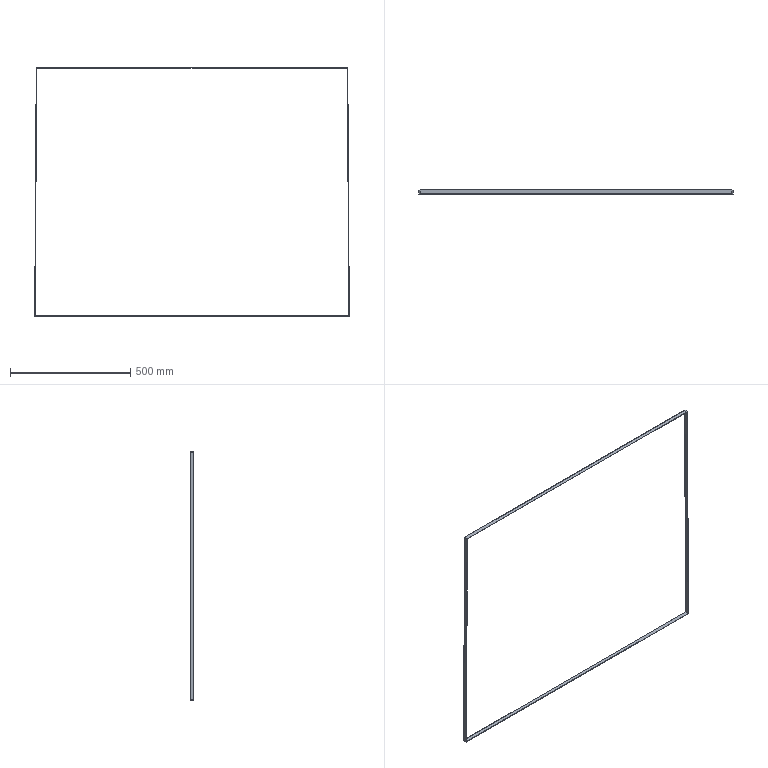Component | NX | LONG_PACKAGING_STRAP | 1 solid | 10 faces | box 1307.7 x 15 x 1031.9 mm | volume 139754 mm3 | plane 10
STEP:
#1=CARTESIAN_POINT('',(0.,0.,0.));
#2=DIRECTION('',(0.,0.,1.));
#3=DIRECTION('',(1.,0.,0.));
#4=AXIS2_PLACEMENT_3D('',#1,#2,#3);
#5=CARTESIAN_POINT('',(-647.456,220.,995.916));
#6=VERTEX_POINT('',#5);
#7=CARTESIAN_POINT('',(647.456,220.,995.916));
#8=VERTEX_POINT('',#7);
#9=CARTESIAN_POINT('',(-645.468,220.,995.916));
#10=DIRECTION('',(1.,0.,0.));
#11=VECTOR('',#10,1.);
#12=LINE('',#9,#11);
#13=CARTESIAN_POINT('',(-645.468,220.,993.916));
#14=DIRECTION('',(0.,1.,0.));
#15=DIRECTION('',(1.,0.,0.));
#16=AXIS2_PLACEMENT_3D('',#13,#14,#15);
#17=PLANE('',#16);
#18=CARTESIAN_POINT('',(0.,-2.));
#19=DIRECTION('',(1.,0.));
#20=VECTOR('',#19,1.);
#21=LINE('',#18,#20);
#22=(GEOMETRIC_REPRESENTATION_CONTEXT(2)PARAMETRIC_REPRESENTATION_CONTEXT()REPRESENTATION_CONTEXT('',''));
#23=DEFINITIONAL_REPRESENTATION('',(#21),#22);
#24=PCURVE('',#17,#23);
#25=CARTESIAN_POINT('',(-645.468,235.,995.916));
#26=DIRECTION('',(0.,0.,-1.));
#27=DIRECTION('',(-1.,0.,0.));
#28=AXIS2_PLACEMENT_3D('',#25,#26,#27);
#29=PLANE('',#28);
#30=CARTESIAN_POINT('',(0.,-15.));
#31=DIRECTION('',(-1.,0.));
#32=VECTOR('',#31,1.);
#33=LINE('',#30,#32);
#34=(GEOMETRIC_REPRESENTATION_CONTEXT(2)PARAMETRIC_REPRESENTATION_CONTEXT()REPRESENTATION_CONTEXT('',''));
#35=DEFINITIONAL_REPRESENTATION('',(#33),#34);
#36=PCURVE('',#29,#35);
#37=SURFACE_CURVE('',#12,(#24,#36),.PCURVE_S1.);
#38=EDGE_CURVE('',#6,#8,#37,.T.);
#39=ORIENTED_EDGE('',*,*,#38,.F.);
#40=CARTESIAN_POINT('',(-653.85,220.,-35.987));
#41=VERTEX_POINT('',#40);
#42=CARTESIAN_POINT('',(-653.838,220.,-33.975));
#43=DIRECTION('',(0.006197,0.,1.));
#44=VECTOR('',#43,1.);
#45=LINE('',#42,#44);
#46=CARTESIAN_POINT('',(-8.37,1027.891));
#47=DIRECTION('',(0.006197,-1.));
#48=VECTOR('',#47,1.);
#49=LINE('',#46,#48);
#50=(GEOMETRIC_REPRESENTATION_CONTEXT(2)PARAMETRIC_REPRESENTATION_CONTEXT()REPRESENTATION_CONTEXT('',''));
#51=DEFINITIONAL_REPRESENTATION('',(#49),#50);
#52=PCURVE('',#17,#51);
#53=CARTESIAN_POINT('',(-653.838,235.,-33.975));
#54=DIRECTION('',(1.,0.,-0.006197));
#55=DIRECTION('',(-0.006197,0.,-1.));
#56=AXIS2_PLACEMENT_3D('',#53,#54,#55);
#57=PLANE('',#56);
#58=CARTESIAN_POINT('',(0.,-15.));
#59=DIRECTION('',(-1.,0.));
#60=VECTOR('',#59,1.);
#61=LINE('',#58,#60);
#62=(GEOMETRIC_REPRESENTATION_CONTEXT(2)PARAMETRIC_REPRESENTATION_CONTEXT()REPRESENTATION_CONTEXT('',''));
#63=DEFINITIONAL_REPRESENTATION('',(#61),#62);
#64=PCURVE('',#57,#63);
#65=SURFACE_CURVE('',#45,(#52,#64),.PCURVE_S1.);
#66=EDGE_CURVE('',#41,#6,#65,.T.);
#67=ORIENTED_EDGE('',*,*,#66,.F.);
#68=CARTESIAN_POINT('',(653.85,220.,-35.987));
#69=VERTEX_POINT('',#68);
#70=CARTESIAN_POINT('',(651.838,220.,-35.987));
#71=DIRECTION('',(-1.,0.,-0.));
#72=VECTOR('',#71,1.);
#73=LINE('',#70,#72);
#74=CARTESIAN_POINT('',(1297.306,1029.903));
#75=DIRECTION('',(-1.,0.));
#76=VECTOR('',#75,1.);
#77=LINE('',#74,#76);
#78=(GEOMETRIC_REPRESENTATION_CONTEXT(2)PARAMETRIC_REPRESENTATION_CONTEXT()REPRESENTATION_CONTEXT('',''));
#79=DEFINITIONAL_REPRESENTATION('',(#77),#78);
#80=PCURVE('',#17,#79);
#81=CARTESIAN_POINT('',(651.838,235.,-35.987));
#82=DIRECTION('',(-0.,0.,1.));
#83=DIRECTION('',(1.,0.,0.));
#84=AXIS2_PLACEMENT_3D('',#81,#82,#83);
#85=PLANE('',#84);
#86=CARTESIAN_POINT('',(0.,-15.));
#87=DIRECTION('',(-1.,0.));
#88=VECTOR('',#87,1.);
#89=LINE('',#86,#88);
#90=(GEOMETRIC_REPRESENTATION_CONTEXT(2)PARAMETRIC_REPRESENTATION_CONTEXT()REPRESENTATION_CONTEXT('',''));
#91=DEFINITIONAL_REPRESENTATION('',(#89),#90);
#92=PCURVE('',#85,#91);
#93=SURFACE_CURVE('',#73,(#80,#92),.PCURVE_S1.);
#94=EDGE_CURVE('',#69,#41,#93,.T.);
#95=ORIENTED_EDGE('',*,*,#94,.F.);
#96=CARTESIAN_POINT('',(647.468,220.,993.928));
#97=DIRECTION('',(0.006197,0.,-1.));
#98=VECTOR('',#97,1.);
#99=LINE('',#96,#98);
#100=CARTESIAN_POINT('',(1292.936,-0.01239));
#101=DIRECTION('',(0.006197,1.));
#102=VECTOR('',#101,1.);
#103=LINE('',#100,#102);
#104=(GEOMETRIC_REPRESENTATION_CONTEXT(2)PARAMETRIC_REPRESENTATION_CONTEXT()REPRESENTATION_CONTEXT('',''));
#105=DEFINITIONAL_REPRESENTATION('',(#103),#104);
#106=PCURVE('',#17,#105);
#107=CARTESIAN_POINT('',(647.468,235.,993.928));
#108=DIRECTION('',(-1.,0.,-0.006197));
#109=DIRECTION('',(-0.006197,0.,1.));
#110=AXIS2_PLACEMENT_3D('',#107,#108,#109);
#111=PLANE('',#110);
#112=CARTESIAN_POINT('',(0.,-15.));
#113=DIRECTION('',(-1.,0.));
#114=VECTOR('',#113,1.);
#115=LINE('',#112,#114);
#116=(GEOMETRIC_REPRESENTATION_CONTEXT(2)PARAMETRIC_REPRESENTATION_CONTEXT()REPRESENTATION_CONTEXT('',''));
#117=DEFINITIONAL_REPRESENTATION('',(#115),#116);
#118=PCURVE('',#111,#117);
#119=SURFACE_CURVE('',#99,(#106,#118),.PCURVE_S1.);
#120=EDGE_CURVE('',#8,#69,#119,.T.);
#121=ORIENTED_EDGE('',*,*,#120,.F.);
#122=EDGE_LOOP('',(#39,#67,#95,#121));
#123=FACE_BOUND('',#122,.T.);
#124=CARTESIAN_POINT('',(-645.468,220.,993.916));
#125=VERTEX_POINT('',#124);
#126=CARTESIAN_POINT('',(645.468,220.,993.916));
#127=VERTEX_POINT('',#126);
#128=CARTESIAN_POINT('',(-645.468,220.,993.916));
#129=DIRECTION('',(1.,0.,0.));
#130=VECTOR('',#129,1.);
#131=LINE('',#128,#130);
#132=CARTESIAN_POINT('',(0.,0.));
#133=DIRECTION('',(1.,0.));
#134=VECTOR('',#133,1.);
#135=LINE('',#132,#134);
#136=(GEOMETRIC_REPRESENTATION_CONTEXT(2)PARAMETRIC_REPRESENTATION_CONTEXT()REPRESENTATION_CONTEXT('',''));
#137=DEFINITIONAL_REPRESENTATION('',(#135),#136);
#138=PCURVE('',#17,#137);
#139=CARTESIAN_POINT('',(-645.468,235.,993.916));
#140=DIRECTION('',(0.,0.,-1.));
#141=DIRECTION('',(-1.,0.,0.));
#142=AXIS2_PLACEMENT_3D('',#139,#140,#141);
#143=PLANE('',#142);
#144=CARTESIAN_POINT('',(0.,-15.));
#145=DIRECTION('',(-1.,0.));
#146=VECTOR('',#145,1.);
#147=LINE('',#144,#146);
#148=(GEOMETRIC_REPRESENTATION_CONTEXT(2)PARAMETRIC_REPRESENTATION_CONTEXT()REPRESENTATION_CONTEXT('',''));
#149=DEFINITIONAL_REPRESENTATION('',(#147),#148);
#150=PCURVE('',#143,#149);
#151=SURFACE_CURVE('',#131,(#138,#150),.PCURVE_S1.);
#152=EDGE_CURVE('',#125,#127,#151,.T.);
#153=ORIENTED_EDGE('',*,*,#152,.T.);
#154=CARTESIAN_POINT('',(651.838,220.,-33.987));
#155=VERTEX_POINT('',#154);
#156=CARTESIAN_POINT('',(645.468,220.,993.916));
#157=DIRECTION('',(0.006197,0.,-1.));
#158=VECTOR('',#157,1.);
#159=LINE('',#156,#158);
#160=CARTESIAN_POINT('',(1290.936,0.));
#161=DIRECTION('',(0.006197,1.));
#162=VECTOR('',#161,1.);
#163=LINE('',#160,#162);
#164=(GEOMETRIC_REPRESENTATION_CONTEXT(2)PARAMETRIC_REPRESENTATION_CONTEXT()REPRESENTATION_CONTEXT('',''));
#165=DEFINITIONAL_REPRESENTATION('',(#163),#164);
#166=PCURVE('',#17,#165);
#167=CARTESIAN_POINT('',(645.468,235.,993.916));
#168=DIRECTION('',(-1.,0.,-0.006197));
#169=DIRECTION('',(-0.006197,0.,1.));
#170=AXIS2_PLACEMENT_3D('',#167,#168,#169);
#171=PLANE('',#170);
#172=CARTESIAN_POINT('',(0.,-15.));
#173=DIRECTION('',(-1.,0.));
#174=VECTOR('',#173,1.);
#175=LINE('',#172,#174);
#176=(GEOMETRIC_REPRESENTATION_CONTEXT(2)PARAMETRIC_REPRESENTATION_CONTEXT()REPRESENTATION_CONTEXT('',''));
#177=DEFINITIONAL_REPRESENTATION('',(#175),#176);
#178=PCURVE('',#171,#177);
#179=SURFACE_CURVE('',#159,(#166,#178),.PCURVE_S1.);
#180=EDGE_CURVE('',#127,#155,#179,.T.);
#181=ORIENTED_EDGE('',*,*,#180,.T.);
#182=CARTESIAN_POINT('',(-651.838,220.,-33.987));
#183=VERTEX_POINT('',#182);
#184=CARTESIAN_POINT('',(651.838,220.,-33.987));
#185=DIRECTION('',(-1.,0.,-0.));
#186=VECTOR('',#185,1.);
#187=LINE('',#184,#186);
#188=CARTESIAN_POINT('',(1297.306,1027.903));
#189=DIRECTION('',(-1.,0.));
#190=VECTOR('',#189,1.);
#191=LINE('',#188,#190);
#192=(GEOMETRIC_REPRESENTATION_CONTEXT(2)PARAMETRIC_REPRESENTATION_CONTEXT()REPRESENTATION_CONTEXT('',''));
#193=DEFINITIONAL_REPRESENTATION('',(#191),#192);
#194=PCURVE('',#17,#193);
#195=CARTESIAN_POINT('',(651.838,235.,-33.987));
#196=DIRECTION('',(-0.,0.,1.));
#197=DIRECTION('',(1.,0.,0.));
#198=AXIS2_PLACEMENT_3D('',#195,#196,#197);
#199=PLANE('',#198);
#200=CARTESIAN_POINT('',(0.,-15.));
#201=DIRECTION('',(-1.,0.));
#202=VECTOR('',#201,1.);
#203=LINE('',#200,#202);
#204=(GEOMETRIC_REPRESENTATION_CONTEXT(2)PARAMETRIC_REPRESENTATION_CONTEXT()REPRESENTATION_CONTEXT('',''));
#205=DEFINITIONAL_REPRESENTATION('',(#203),#204);
#206=PCURVE('',#199,#205);
#207=SURFACE_CURVE('',#187,(#194,#206),.PCURVE_S1.);
#208=EDGE_CURVE('',#155,#183,#207,.T.);
#209=ORIENTED_EDGE('',*,*,#208,.T.);
#210=CARTESIAN_POINT('',(-651.838,220.,-33.987));
#211=DIRECTION('',(0.006197,0.,1.));
#212=VECTOR('',#211,1.);
#213=LINE('',#210,#212);
#214=CARTESIAN_POINT('',(-6.37,1027.903));
#215=DIRECTION('',(0.006197,-1.));
#216=VECTOR('',#215,1.);
#217=LINE('',#214,#216);
#218=(GEOMETRIC_REPRESENTATION_CONTEXT(2)PARAMETRIC_REPRESENTATION_CONTEXT()REPRESENTATION_CONTEXT('',''));
#219=DEFINITIONAL_REPRESENTATION('',(#217),#218);
#220=PCURVE('',#17,#219);
#221=CARTESIAN_POINT('',(-651.838,235.,-33.987));
#222=DIRECTION('',(1.,0.,-0.006197));
#223=DIRECTION('',(-0.006197,0.,-1.));
#224=AXIS2_PLACEMENT_3D('',#221,#222,#223);
#225=PLANE('',#224);
#226=CARTESIAN_POINT('',(0.,-15.));
#227=DIRECTION('',(-1.,0.));
#228=VECTOR('',#227,1.);
#229=LINE('',#226,#228);
#230=(GEOMETRIC_REPRESENTATION_CONTEXT(2)PARAMETRIC_REPRESENTATION_CONTEXT()REPRESENTATION_CONTEXT('',''));
#231=DEFINITIONAL_REPRESENTATION('',(#229),#230);
#232=PCURVE('',#225,#231);
#233=SURFACE_CURVE('',#213,(#220,#232),.PCURVE_S1.);
#234=EDGE_CURVE('',#183,#125,#233,.T.);
#235=ORIENTED_EDGE('',*,*,#234,.T.);
#236=EDGE_LOOP('',(#153,#181,#209,#235));
#237=FACE_BOUND('',#236,.T.);
#238=ADVANCED_FACE('',(#123,#237),#17,.F.);
#239=CARTESIAN_POINT('',(653.85,235.,-35.987));
#240=VERTEX_POINT('',#239);
#241=CARTESIAN_POINT('',(-653.85,235.,-35.987));
#242=VERTEX_POINT('',#241);
#243=CARTESIAN_POINT('',(651.838,235.,-35.987));
#244=DIRECTION('',(-1.,0.,-0.));
#245=VECTOR('',#244,1.);
#246=LINE('',#243,#245);
#247=CARTESIAN_POINT('',(651.838,235.,-33.987));
#248=DIRECTION('',(0.,1.,0.));
#249=DIRECTION('',(-1.,0.,-0.));
#250=AXIS2_PLACEMENT_3D('',#247,#248,#249);
#251=PLANE('',#250);
#252=CARTESIAN_POINT('',(0.,-2.));
#253=DIRECTION('',(1.,-0.));
#254=VECTOR('',#253,1.);
#255=LINE('',#252,#254);
#256=(GEOMETRIC_REPRESENTATION_CONTEXT(2)PARAMETRIC_REPRESENTATION_CONTEXT()REPRESENTATION_CONTEXT('',''));
#257=DEFINITIONAL_REPRESENTATION('',(#255),#256);
#258=PCURVE('',#251,#257);
#259=CARTESIAN_POINT('',(0.,0.));
#260=DIRECTION('',(-1.,0.));
#261=VECTOR('',#260,1.);
#262=LINE('',#259,#261);
#263=(GEOMETRIC_REPRESENTATION_CONTEXT(2)PARAMETRIC_REPRESENTATION_CONTEXT()REPRESENTATION_CONTEXT('',''));
#264=DEFINITIONAL_REPRESENTATION('',(#262),#263);
#265=PCURVE('',#85,#264);
#266=SURFACE_CURVE('',#246,(#258,#265),.PCURVE_S1.);
#267=EDGE_CURVE('',#240,#242,#266,.T.);
#268=ORIENTED_EDGE('',*,*,#267,.T.);
#269=CARTESIAN_POINT('',(-647.456,235.,995.916));
#270=VERTEX_POINT('',#269);
#271=CARTESIAN_POINT('',(-653.838,235.,-33.975));
#272=DIRECTION('',(0.006197,0.,1.));
#273=VECTOR('',#272,1.);
#274=LINE('',#271,#273);
#275=CARTESIAN_POINT('',(1305.676,0.01239));
#276=DIRECTION('',(-0.006197,1.));
#277=VECTOR('',#276,1.);
#278=LINE('',#275,#277);
#279=(GEOMETRIC_REPRESENTATION_CONTEXT(2)PARAMETRIC_REPRESENTATION_CONTEXT()REPRESENTATION_CONTEXT('',''));
#280=DEFINITIONAL_REPRESENTATION('',(#278),#279);
#281=PCURVE('',#251,#280);
#282=CARTESIAN_POINT('',(0.,0.));
#283=DIRECTION('',(-1.,0.));
#284=VECTOR('',#283,1.);
#285=LINE('',#282,#284);
#286=(GEOMETRIC_REPRESENTATION_CONTEXT(2)PARAMETRIC_REPRESENTATION_CONTEXT()REPRESENTATION_CONTEXT('',''));
#287=DEFINITIONAL_REPRESENTATION('',(#285),#286);
#288=PCURVE('',#57,#287);
#289=SURFACE_CURVE('',#274,(#281,#288),.PCURVE_S1.);
#290=EDGE_CURVE('',#242,#270,#289,.T.);
#291=ORIENTED_EDGE('',*,*,#290,.T.);
#292=CARTESIAN_POINT('',(647.456,235.,995.916));
#293=VERTEX_POINT('',#292);
#294=CARTESIAN_POINT('',(-645.468,235.,995.916));
#295=DIRECTION('',(1.,0.,0.));
#296=VECTOR('',#295,1.);
#297=LINE('',#294,#296);
#298=CARTESIAN_POINT('',(1297.306,1029.903));
#299=DIRECTION('',(-1.,-0.));
#300=VECTOR('',#299,1.);
#301=LINE('',#298,#300);
#302=(GEOMETRIC_REPRESENTATION_CONTEXT(2)PARAMETRIC_REPRESENTATION_CONTEXT()REPRESENTATION_CONTEXT('',''));
#303=DEFINITIONAL_REPRESENTATION('',(#301),#302);
#304=PCURVE('',#251,#303);
#305=CARTESIAN_POINT('',(0.,0.));
#306=DIRECTION('',(-1.,0.));
#307=VECTOR('',#306,1.);
#308=LINE('',#305,#307);
#309=(GEOMETRIC_REPRESENTATION_CONTEXT(2)PARAMETRIC_REPRESENTATION_CONTEXT()REPRESENTATION_CONTEXT('',''));
#310=DEFINITIONAL_REPRESENTATION('',(#308),#309);
#311=PCURVE('',#29,#310);
#312=SURFACE_CURVE('',#297,(#304,#311),.PCURVE_S1.);
#313=EDGE_CURVE('',#270,#293,#312,.T.);
#314=ORIENTED_EDGE('',*,*,#313,.T.);
#315=CARTESIAN_POINT('',(647.468,235.,993.928));
#316=DIRECTION('',(0.006197,0.,-1.));
#317=VECTOR('',#316,1.);
#318=LINE('',#315,#317);
#319=CARTESIAN_POINT('',(4.37,1027.915));
#320=DIRECTION('',(-0.006197,-1.));
#321=VECTOR('',#320,1.);
#322=LINE('',#319,#321);
#323=(GEOMETRIC_REPRESENTATION_CONTEXT(2)PARAMETRIC_REPRESENTATION_CONTEXT()REPRESENTATION_CONTEXT('',''));
#324=DEFINITIONAL_REPRESENTATION('',(#322),#323);
#325=PCURVE('',#251,#324);
#326=CARTESIAN_POINT('',(0.,0.));
#327=DIRECTION('',(-1.,0.));
#328=VECTOR('',#327,1.);
#329=LINE('',#326,#328);
#330=(GEOMETRIC_REPRESENTATION_CONTEXT(2)PARAMETRIC_REPRESENTATION_CONTEXT()REPRESENTATION_CONTEXT('',''));
#331=DEFINITIONAL_REPRESENTATION('',(#329),#330);
#332=PCURVE('',#111,#331);
#333=SURFACE_CURVE('',#318,(#325,#332),.PCURVE_S1.);
#334=EDGE_CURVE('',#293,#240,#333,.T.);
#335=ORIENTED_EDGE('',*,*,#334,.T.);
#336=EDGE_LOOP('',(#268,#291,#314,#335));
#337=FACE_BOUND('',#336,.T.);
#338=CARTESIAN_POINT('',(651.838,235.,-33.987));
#339=VERTEX_POINT('',#338);
#340=CARTESIAN_POINT('',(-651.838,235.,-33.987));
#341=VERTEX_POINT('',#340);
#342=CARTESIAN_POINT('',(651.838,235.,-33.987));
#343=DIRECTION('',(-1.,0.,-0.));
#344=VECTOR('',#343,1.);
#345=LINE('',#342,#344);
#346=CARTESIAN_POINT('',(0.,0.));
#347=DIRECTION('',(1.,-0.));
#348=VECTOR('',#347,1.);
#349=LINE('',#346,#348);
#350=(GEOMETRIC_REPRESENTATION_CONTEXT(2)PARAMETRIC_REPRESENTATION_CONTEXT()REPRESENTATION_CONTEXT('',''));
#351=DEFINITIONAL_REPRESENTATION('',(#349),#350);
#352=PCURVE('',#251,#351);
#353=CARTESIAN_POINT('',(0.,0.));
#354=DIRECTION('',(-1.,0.));
#355=VECTOR('',#354,1.);
#356=LINE('',#353,#355);
#357=(GEOMETRIC_REPRESENTATION_CONTEXT(2)PARAMETRIC_REPRESENTATION_CONTEXT()REPRESENTATION_CONTEXT('',''));
#358=DEFINITIONAL_REPRESENTATION('',(#356),#357);
#359=PCURVE('',#199,#358);
#360=SURFACE_CURVE('',#345,(#352,#359),.PCURVE_S1.);
#361=EDGE_CURVE('',#339,#341,#360,.T.);
#362=ORIENTED_EDGE('',*,*,#361,.F.);
#363=CARTESIAN_POINT('',(645.468,235.,993.916));
#364=VERTEX_POINT('',#363);
#365=CARTESIAN_POINT('',(645.468,235.,993.916));
#366=DIRECTION('',(0.006197,0.,-1.));
#367=VECTOR('',#366,1.);
#368=LINE('',#365,#367);
#369=CARTESIAN_POINT('',(6.37,1027.903));
#370=DIRECTION('',(-0.006197,-1.));
#371=VECTOR('',#370,1.);
#372=LINE('',#369,#371);
#373=(GEOMETRIC_REPRESENTATION_CONTEXT(2)PARAMETRIC_REPRESENTATION_CONTEXT()REPRESENTATION_CONTEXT('',''));
#374=DEFINITIONAL_REPRESENTATION('',(#372),#373);
#375=PCURVE('',#251,#374);
#376=CARTESIAN_POINT('',(0.,0.));
#377=DIRECTION('',(-1.,0.));
#378=VECTOR('',#377,1.);
#379=LINE('',#376,#378);
#380=(GEOMETRIC_REPRESENTATION_CONTEXT(2)PARAMETRIC_REPRESENTATION_CONTEXT()REPRESENTATION_CONTEXT('',''));
#381=DEFINITIONAL_REPRESENTATION('',(#379),#380);
#382=PCURVE('',#171,#381);
#383=SURFACE_CURVE('',#368,(#375,#382),.PCURVE_S1.);
#384=EDGE_CURVE('',#364,#339,#383,.T.);
#385=ORIENTED_EDGE('',*,*,#384,.F.);
#386=CARTESIAN_POINT('',(-645.468,235.,993.916));
#387=VERTEX_POINT('',#386);
#388=CARTESIAN_POINT('',(-645.468,235.,993.916));
#389=DIRECTION('',(1.,0.,0.));
#390=VECTOR('',#389,1.);
#391=LINE('',#388,#390);
#392=CARTESIAN_POINT('',(1297.306,1027.903));
#393=DIRECTION('',(-1.,-0.));
#394=VECTOR('',#393,1.);
#395=LINE('',#392,#394);
#396=(GEOMETRIC_REPRESENTATION_CONTEXT(2)PARAMETRIC_REPRESENTATION_CONTEXT()REPRESENTATION_CONTEXT('',''));
#397=DEFINITIONAL_REPRESENTATION('',(#395),#396);
#398=PCURVE('',#251,#397);
#399=CARTESIAN_POINT('',(0.,0.));
#400=DIRECTION('',(-1.,0.));
#401=VECTOR('',#400,1.);
#402=LINE('',#399,#401);
#403=(GEOMETRIC_REPRESENTATION_CONTEXT(2)PARAMETRIC_REPRESENTATION_CONTEXT()REPRESENTATION_CONTEXT('',''));
#404=DEFINITIONAL_REPRESENTATION('',(#402),#403);
#405=PCURVE('',#143,#404);
#406=SURFACE_CURVE('',#391,(#398,#405),.PCURVE_S1.);
#407=EDGE_CURVE('',#387,#364,#406,.T.);
#408=ORIENTED_EDGE('',*,*,#407,.F.);
#409=CARTESIAN_POINT('',(-651.838,235.,-33.987));
#410=DIRECTION('',(0.006197,0.,1.));
#411=VECTOR('',#410,1.);
#412=LINE('',#409,#411);
#413=CARTESIAN_POINT('',(1303.676,-0.));
#414=DIRECTION('',(-0.006197,1.));
#415=VECTOR('',#414,1.);
#416=LINE('',#413,#415);
#417=(GEOMETRIC_REPRESENTATION_CONTEXT(2)PARAMETRIC_REPRESENTATION_CONTEXT()REPRESENTATION_CONTEXT('',''));
#418=DEFINITIONAL_REPRESENTATION('',(#416),#417);
#419=PCURVE('',#251,#418);
#420=CARTESIAN_POINT('',(0.,0.));
#421=DIRECTION('',(-1.,0.));
#422=VECTOR('',#421,1.);
#423=LINE('',#420,#422);
#424=(GEOMETRIC_REPRESENTATION_CONTEXT(2)PARAMETRIC_REPRESENTATION_CONTEXT()REPRESENTATION_CONTEXT('',''));
#425=DEFINITIONAL_REPRESENTATION('',(#423),#424);
#426=PCURVE('',#225,#425);
#427=SURFACE_CURVE('',#412,(#419,#426),.PCURVE_S1.);
#428=EDGE_CURVE('',#341,#387,#427,.T.);
#429=ORIENTED_EDGE('',*,*,#428,.F.);
#430=EDGE_LOOP('',(#362,#385,#408,#429));
#431=FACE_BOUND('',#430,.T.);
#432=ADVANCED_FACE('',(#337,#431),#251,.T.);
#433=ORIENTED_EDGE('',*,*,#66,.T.);
#434=CARTESIAN_POINT('',(-647.456,235.,995.916));
#435=DIRECTION('',(0.,-1.,0.));
#436=VECTOR('',#435,1.);
#437=LINE('',#434,#436);
#438=CARTESIAN_POINT('',(-1029.91,0.));
#439=DIRECTION('',(0.,-1.));
#440=VECTOR('',#439,1.);
#441=LINE('',#438,#440);
#442=(GEOMETRIC_REPRESENTATION_CONTEXT(2)PARAMETRIC_REPRESENTATION_CONTEXT()REPRESENTATION_CONTEXT('',''));
#443=DEFINITIONAL_REPRESENTATION('',(#441),#442);
#444=PCURVE('',#57,#443);
#445=CARTESIAN_POINT('',(1.988,0.));
#446=DIRECTION('',(0.,-1.));
#447=VECTOR('',#446,1.);
#448=LINE('',#445,#447);
#449=(GEOMETRIC_REPRESENTATION_CONTEXT(2)PARAMETRIC_REPRESENTATION_CONTEXT()REPRESENTATION_CONTEXT('',''));
#450=DEFINITIONAL_REPRESENTATION('',(#448),#449);
#451=PCURVE('',#29,#450);
#452=SURFACE_CURVE('',#437,(#444,#451),.PCURVE_S1.);
#453=EDGE_CURVE('',#270,#6,#452,.T.);
#454=ORIENTED_EDGE('',*,*,#453,.F.);
#455=ORIENTED_EDGE('',*,*,#290,.F.);
#456=CARTESIAN_POINT('',(-653.85,235.,-35.987));
#457=DIRECTION('',(0.,-1.,0.));
#458=VECTOR('',#457,1.);
#459=LINE('',#456,#458);
#460=CARTESIAN_POINT('',(2.012,0.));
#461=DIRECTION('',(0.,-1.));
#462=VECTOR('',#461,1.);
#463=LINE('',#460,#462);
#464=(GEOMETRIC_REPRESENTATION_CONTEXT(2)PARAMETRIC_REPRESENTATION_CONTEXT()REPRESENTATION_CONTEXT('',''));
#465=DEFINITIONAL_REPRESENTATION('',(#463),#464);
#466=PCURVE('',#57,#465);
#467=CARTESIAN_POINT('',(-1305.689,0.));
#468=DIRECTION('',(0.,-1.));
#469=VECTOR('',#468,1.);
#470=LINE('',#467,#469);
#471=(GEOMETRIC_REPRESENTATION_CONTEXT(2)PARAMETRIC_REPRESENTATION_CONTEXT()REPRESENTATION_CONTEXT('',''));
#472=DEFINITIONAL_REPRESENTATION('',(#470),#471);
#473=PCURVE('',#85,#472);
#474=SURFACE_CURVE('',#459,(#466,#473),.PCURVE_S1.);
#475=EDGE_CURVE('',#242,#41,#474,.T.);
#476=ORIENTED_EDGE('',*,*,#475,.T.);
#477=EDGE_LOOP('',(#433,#454,#455,#476));
#478=FACE_BOUND('',#477,.T.);
#479=ADVANCED_FACE('',(#478),#57,.F.);
#480=ORIENTED_EDGE('',*,*,#38,.T.);
#481=CARTESIAN_POINT('',(647.456,235.,995.916));
#482=DIRECTION('',(0.,-1.,0.));
#483=VECTOR('',#482,1.);
#484=LINE('',#481,#483);
#485=CARTESIAN_POINT('',(-1292.924,0.));
#486=DIRECTION('',(0.,-1.));
#487=VECTOR('',#486,1.);
#488=LINE('',#485,#487);
#489=(GEOMETRIC_REPRESENTATION_CONTEXT(2)PARAMETRIC_REPRESENTATION_CONTEXT()REPRESENTATION_CONTEXT('',''));
#490=DEFINITIONAL_REPRESENTATION('',(#488),#489);
#491=PCURVE('',#29,#490);
#492=CARTESIAN_POINT('',(1.988,0.));
#493=DIRECTION('',(0.,-1.));
#494=VECTOR('',#493,1.);
#495=LINE('',#492,#494);
#496=(GEOMETRIC_REPRESENTATION_CONTEXT(2)PARAMETRIC_REPRESENTATION_CONTEXT()REPRESENTATION_CONTEXT('',''));
#497=DEFINITIONAL_REPRESENTATION('',(#495),#496);
#498=PCURVE('',#111,#497);
#499=SURFACE_CURVE('',#484,(#491,#498),.PCURVE_S1.);
#500=EDGE_CURVE('',#293,#8,#499,.T.);
#501=ORIENTED_EDGE('',*,*,#500,.F.);
#502=ORIENTED_EDGE('',*,*,#313,.F.);
#503=ORIENTED_EDGE('',*,*,#453,.T.);
#504=EDGE_LOOP('',(#480,#501,#502,#503));
#505=FACE_BOUND('',#504,.T.);
#506=ADVANCED_FACE('',(#505),#29,.F.);
#507=ORIENTED_EDGE('',*,*,#120,.T.);
#508=CARTESIAN_POINT('',(653.85,235.,-35.987));
#509=DIRECTION('',(0.,-1.,0.));
#510=VECTOR('',#509,1.);
#511=LINE('',#508,#510);
#512=CARTESIAN_POINT('',(-1029.935,0.));
#513=DIRECTION('',(0.,-1.));
#514=VECTOR('',#513,1.);
#515=LINE('',#512,#514);
#516=(GEOMETRIC_REPRESENTATION_CONTEXT(2)PARAMETRIC_REPRESENTATION_CONTEXT()REPRESENTATION_CONTEXT('',''));
#517=DEFINITIONAL_REPRESENTATION('',(#515),#516);
#518=PCURVE('',#111,#517);
#519=CARTESIAN_POINT('',(2.012,0.));
#520=DIRECTION('',(0.,-1.));
#521=VECTOR('',#520,1.);
#522=LINE('',#519,#521);
#523=(GEOMETRIC_REPRESENTATION_CONTEXT(2)PARAMETRIC_REPRESENTATION_CONTEXT()REPRESENTATION_CONTEXT('',''));
#524=DEFINITIONAL_REPRESENTATION('',(#522),#523);
#525=PCURVE('',#85,#524);
#526=SURFACE_CURVE('',#511,(#518,#525),.PCURVE_S1.);
#527=EDGE_CURVE('',#240,#69,#526,.T.);
#528=ORIENTED_EDGE('',*,*,#527,.F.);
#529=ORIENTED_EDGE('',*,*,#334,.F.);
#530=ORIENTED_EDGE('',*,*,#500,.T.);
#531=EDGE_LOOP('',(#507,#528,#529,#530));
#532=FACE_BOUND('',#531,.T.);
#533=ADVANCED_FACE('',(#532),#111,.F.);
#534=ORIENTED_EDGE('',*,*,#94,.T.);
#535=ORIENTED_EDGE('',*,*,#475,.F.);
#536=ORIENTED_EDGE('',*,*,#267,.F.);
#537=ORIENTED_EDGE('',*,*,#527,.T.);
#538=EDGE_LOOP('',(#534,#535,#536,#537));
#539=FACE_BOUND('',#538,.T.);
#540=ADVANCED_FACE('',(#539),#85,.F.);
#541=ORIENTED_EDGE('',*,*,#234,.F.);
#542=CARTESIAN_POINT('',(-651.838,235.,-33.987));
#543=DIRECTION('',(0.,-1.,0.));
#544=VECTOR('',#543,1.);
#545=LINE('',#542,#544);
#546=CARTESIAN_POINT('',(0.,0.));
#547=DIRECTION('',(0.,-1.));
#548=VECTOR('',#547,1.);
#549=LINE('',#546,#548);
#550=(GEOMETRIC_REPRESENTATION_CONTEXT(2)PARAMETRIC_REPRESENTATION_CONTEXT()REPRESENTATION_CONTEXT('',''));
#551=DEFINITIONAL_REPRESENTATION('',(#549),#550);
#552=PCURVE('',#225,#551);
#553=CARTESIAN_POINT('',(-1303.676,0.));
#554=DIRECTION('',(0.,-1.));
#555=VECTOR('',#554,1.);
#556=LINE('',#553,#555);
#557=(GEOMETRIC_REPRESENTATION_CONTEXT(2)PARAMETRIC_REPRESENTATION_CONTEXT()REPRESENTATION_CONTEXT('',''));
#558=DEFINITIONAL_REPRESENTATION('',(#556),#557);
#559=PCURVE('',#199,#558);
#560=SURFACE_CURVE('',#545,(#552,#559),.PCURVE_S1.);
#561=EDGE_CURVE('',#341,#183,#560,.T.);
#562=ORIENTED_EDGE('',*,*,#561,.F.);
#563=ORIENTED_EDGE('',*,*,#428,.T.);
#564=CARTESIAN_POINT('',(-645.468,235.,993.916));
#565=DIRECTION('',(0.,-1.,0.));
#566=VECTOR('',#565,1.);
#567=LINE('',#564,#566);
#568=CARTESIAN_POINT('',(-1027.923,0.));
#569=DIRECTION('',(0.,-1.));
#570=VECTOR('',#569,1.);
#571=LINE('',#568,#570);
#572=(GEOMETRIC_REPRESENTATION_CONTEXT(2)PARAMETRIC_REPRESENTATION_CONTEXT()REPRESENTATION_CONTEXT('',''));
#573=DEFINITIONAL_REPRESENTATION('',(#571),#572);
#574=PCURVE('',#225,#573);
#575=CARTESIAN_POINT('',(0.,0.));
#576=DIRECTION('',(0.,-1.));
#577=VECTOR('',#576,1.);
#578=LINE('',#575,#577);
#579=(GEOMETRIC_REPRESENTATION_CONTEXT(2)PARAMETRIC_REPRESENTATION_CONTEXT()REPRESENTATION_CONTEXT('',''));
#580=DEFINITIONAL_REPRESENTATION('',(#578),#579);
#581=PCURVE('',#143,#580);
#582=SURFACE_CURVE('',#567,(#574,#581),.PCURVE_S1.);
#583=EDGE_CURVE('',#387,#125,#582,.T.);
#584=ORIENTED_EDGE('',*,*,#583,.T.);
#585=EDGE_LOOP('',(#541,#562,#563,#584));
#586=FACE_BOUND('',#585,.T.);
#587=ADVANCED_FACE('',(#586),#225,.T.);
#588=ORIENTED_EDGE('',*,*,#152,.F.);
#589=ORIENTED_EDGE('',*,*,#583,.F.);
#590=ORIENTED_EDGE('',*,*,#407,.T.);
#591=CARTESIAN_POINT('',(645.468,235.,993.916));
#592=DIRECTION('',(0.,-1.,0.));
#593=VECTOR('',#592,1.);
#594=LINE('',#591,#593);
#595=CARTESIAN_POINT('',(-1290.936,0.));
#596=DIRECTION('',(0.,-1.));
#597=VECTOR('',#596,1.);
#598=LINE('',#595,#597);
#599=(GEOMETRIC_REPRESENTATION_CONTEXT(2)PARAMETRIC_REPRESENTATION_CONTEXT()REPRESENTATION_CONTEXT('',''));
#600=DEFINITIONAL_REPRESENTATION('',(#598),#599);
#601=PCURVE('',#143,#600);
#602=CARTESIAN_POINT('',(0.,0.));
#603=DIRECTION('',(0.,-1.));
#604=VECTOR('',#603,1.);
#605=LINE('',#602,#604);
#606=(GEOMETRIC_REPRESENTATION_CONTEXT(2)PARAMETRIC_REPRESENTATION_CONTEXT()REPRESENTATION_CONTEXT('',''));
#607=DEFINITIONAL_REPRESENTATION('',(#605),#606);
#608=PCURVE('',#171,#607);
#609=SURFACE_CURVE('',#594,(#601,#608),.PCURVE_S1.);
#610=EDGE_CURVE('',#364,#127,#609,.T.);
#611=ORIENTED_EDGE('',*,*,#610,.T.);
#612=EDGE_LOOP('',(#588,#589,#590,#611));
#613=FACE_BOUND('',#612,.T.);
#614=ADVANCED_FACE('',(#613),#143,.T.);
#615=ORIENTED_EDGE('',*,*,#180,.F.);
#616=ORIENTED_EDGE('',*,*,#610,.F.);
#617=ORIENTED_EDGE('',*,*,#384,.T.);
#618=CARTESIAN_POINT('',(651.838,235.,-33.987));
#619=DIRECTION('',(0.,-1.,0.));
#620=VECTOR('',#619,1.);
#621=LINE('',#618,#620);
#622=CARTESIAN_POINT('',(-1027.923,0.));
#623=DIRECTION('',(0.,-1.));
#624=VECTOR('',#623,1.);
#625=LINE('',#622,#624);
#626=(GEOMETRIC_REPRESENTATION_CONTEXT(2)PARAMETRIC_REPRESENTATION_CONTEXT()REPRESENTATION_CONTEXT('',''));
#627=DEFINITIONAL_REPRESENTATION('',(#625),#626);
#628=PCURVE('',#171,#627);
#629=CARTESIAN_POINT('',(0.,0.));
#630=DIRECTION('',(0.,-1.));
#631=VECTOR('',#630,1.);
#632=LINE('',#629,#631);
#633=(GEOMETRIC_REPRESENTATION_CONTEXT(2)PARAMETRIC_REPRESENTATION_CONTEXT()REPRESENTATION_CONTEXT('',''));
#634=DEFINITIONAL_REPRESENTATION('',(#632),#633);
#635=PCURVE('',#199,#634);
#636=SURFACE_CURVE('',#621,(#628,#635),.PCURVE_S1.);
#637=EDGE_CURVE('',#339,#155,#636,.T.);
#638=ORIENTED_EDGE('',*,*,#637,.T.);
#639=EDGE_LOOP('',(#615,#616,#617,#638));
#640=FACE_BOUND('',#639,.T.);
#641=ADVANCED_FACE('',(#640),#171,.T.);
#642=ORIENTED_EDGE('',*,*,#208,.F.);
#643=ORIENTED_EDGE('',*,*,#637,.F.);
#644=ORIENTED_EDGE('',*,*,#361,.T.);
#645=ORIENTED_EDGE('',*,*,#561,.T.);
#646=EDGE_LOOP('',(#642,#643,#644,#645));
#647=FACE_BOUND('',#646,.T.);
#648=ADVANCED_FACE('',(#647),#199,.T.);
#649=CLOSED_SHELL('',(#238,#432,#479,#506,#533,#540,#587,#614,#641,#648));
#650=MANIFOLD_SOLID_BREP('',#649);
#651=(LENGTH_UNIT()NAMED_UNIT(*)SI_UNIT(.MILLI.,.METRE.));
#652=UNCERTAINTY_MEASURE_WITH_UNIT(LENGTH_MEASURE(0.0000001),#651,'','');
#653=(NAMED_UNIT(*)PLANE_ANGLE_UNIT()SI_UNIT($,.RADIAN.));
#654=(NAMED_UNIT(*)SI_UNIT($,.STERADIAN.)SOLID_ANGLE_UNIT());
#655=(GEOMETRIC_REPRESENTATION_CONTEXT(3)GLOBAL_UNCERTAINTY_ASSIGNED_CONTEXT((#652))GLOBAL_UNIT_ASSIGNED_CONTEXT((#651,#653,#654))REPRESENTATION_CONTEXT('',''));
#656=ADVANCED_BREP_SHAPE_REPRESENTATION('',(#4,#650),#655);